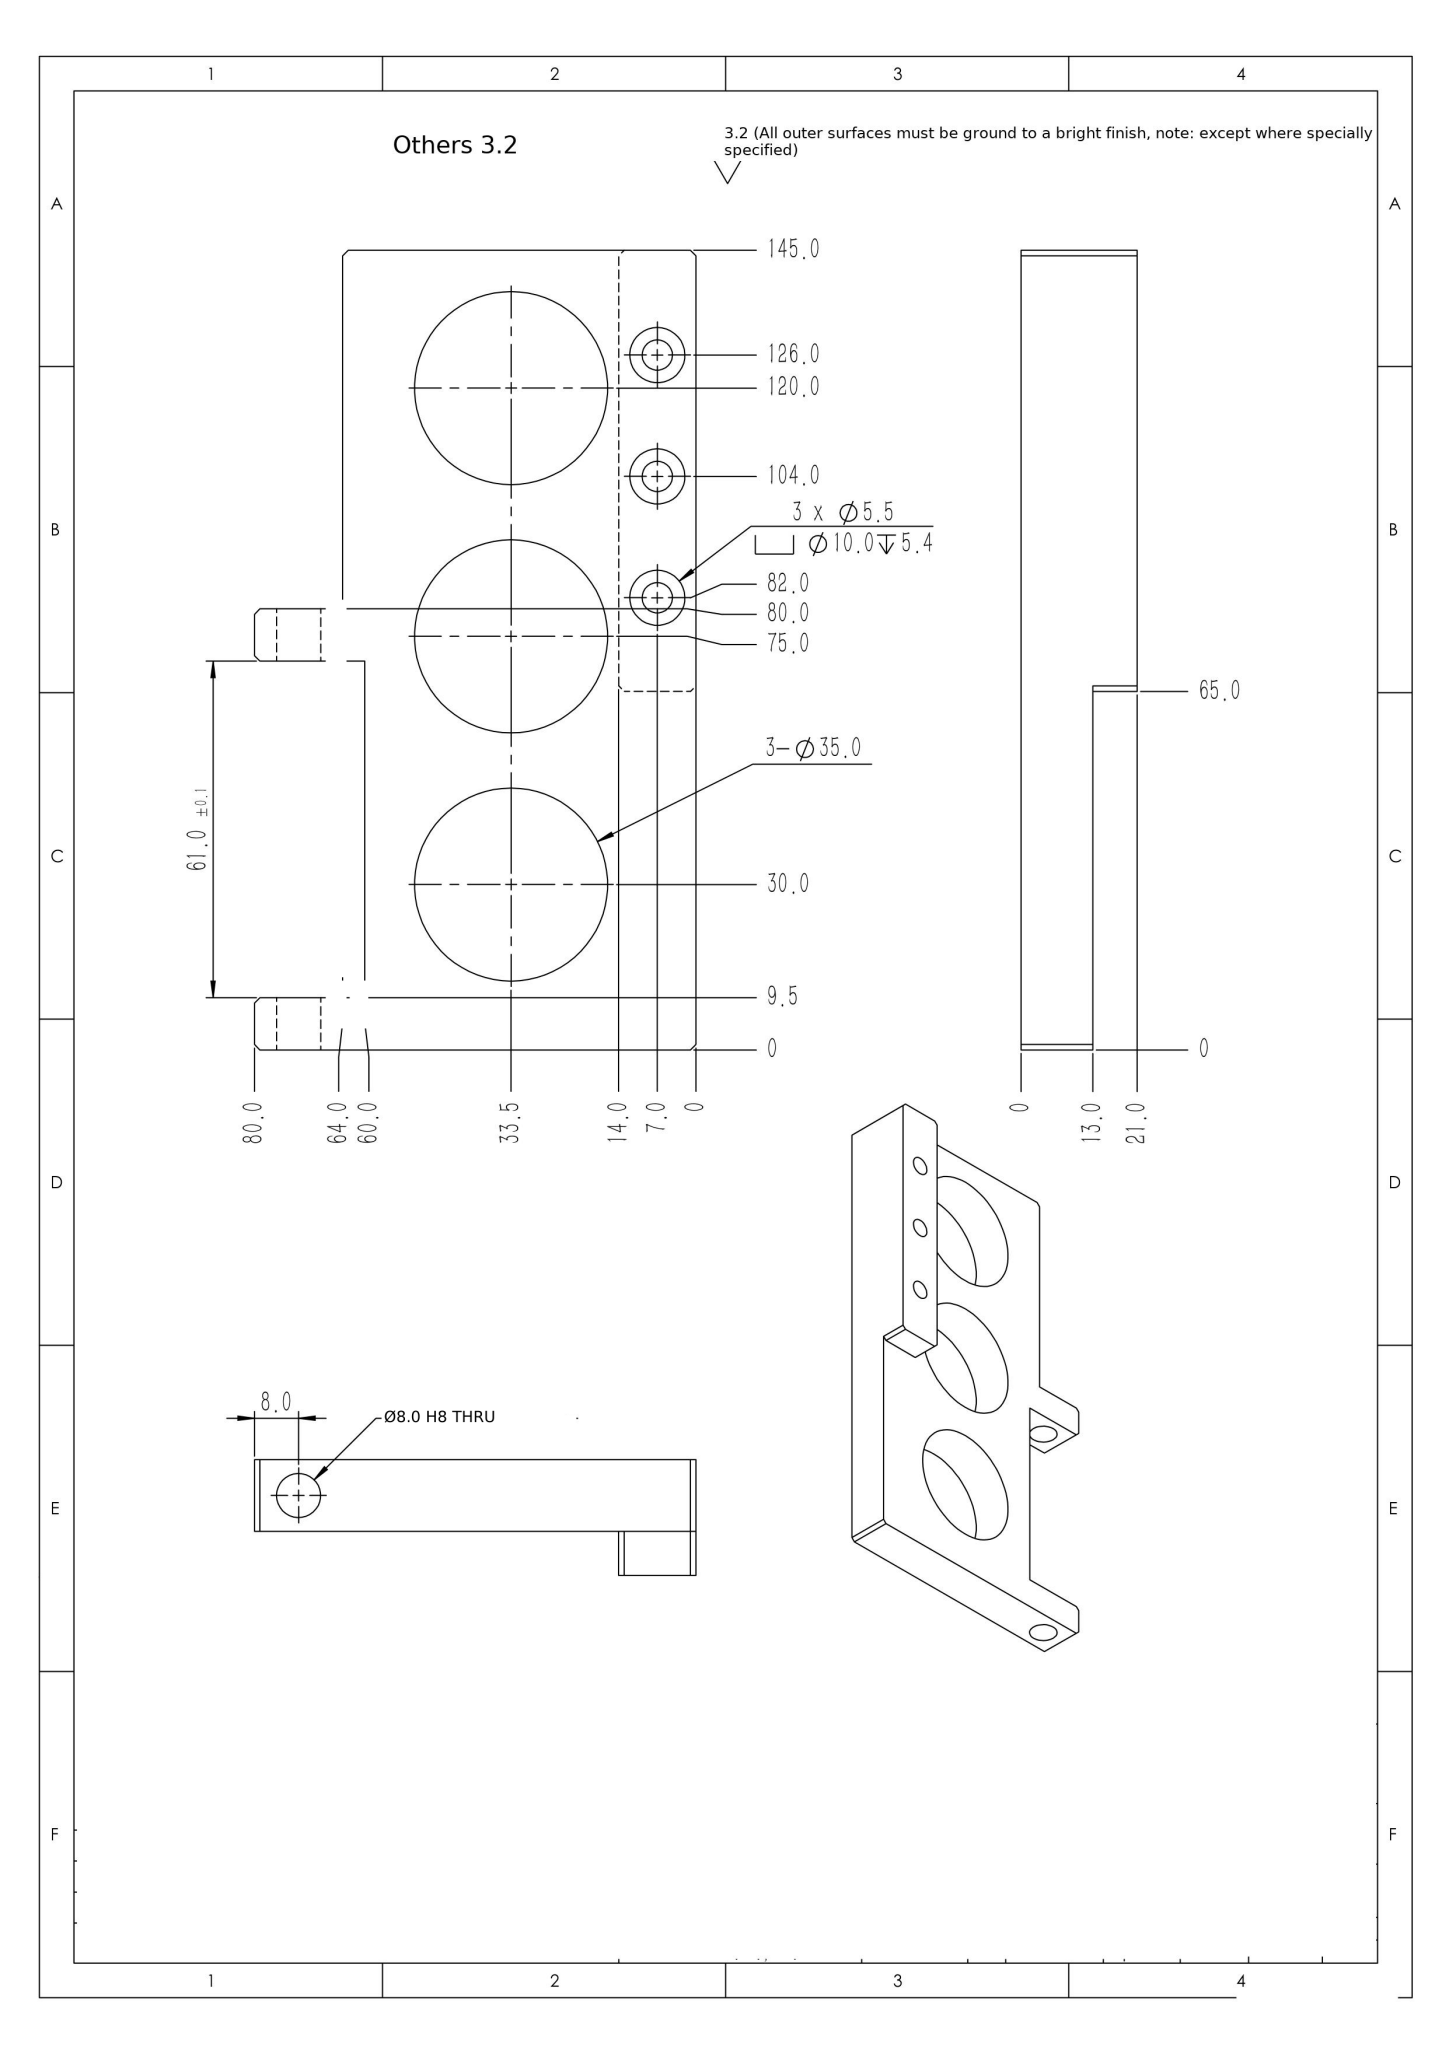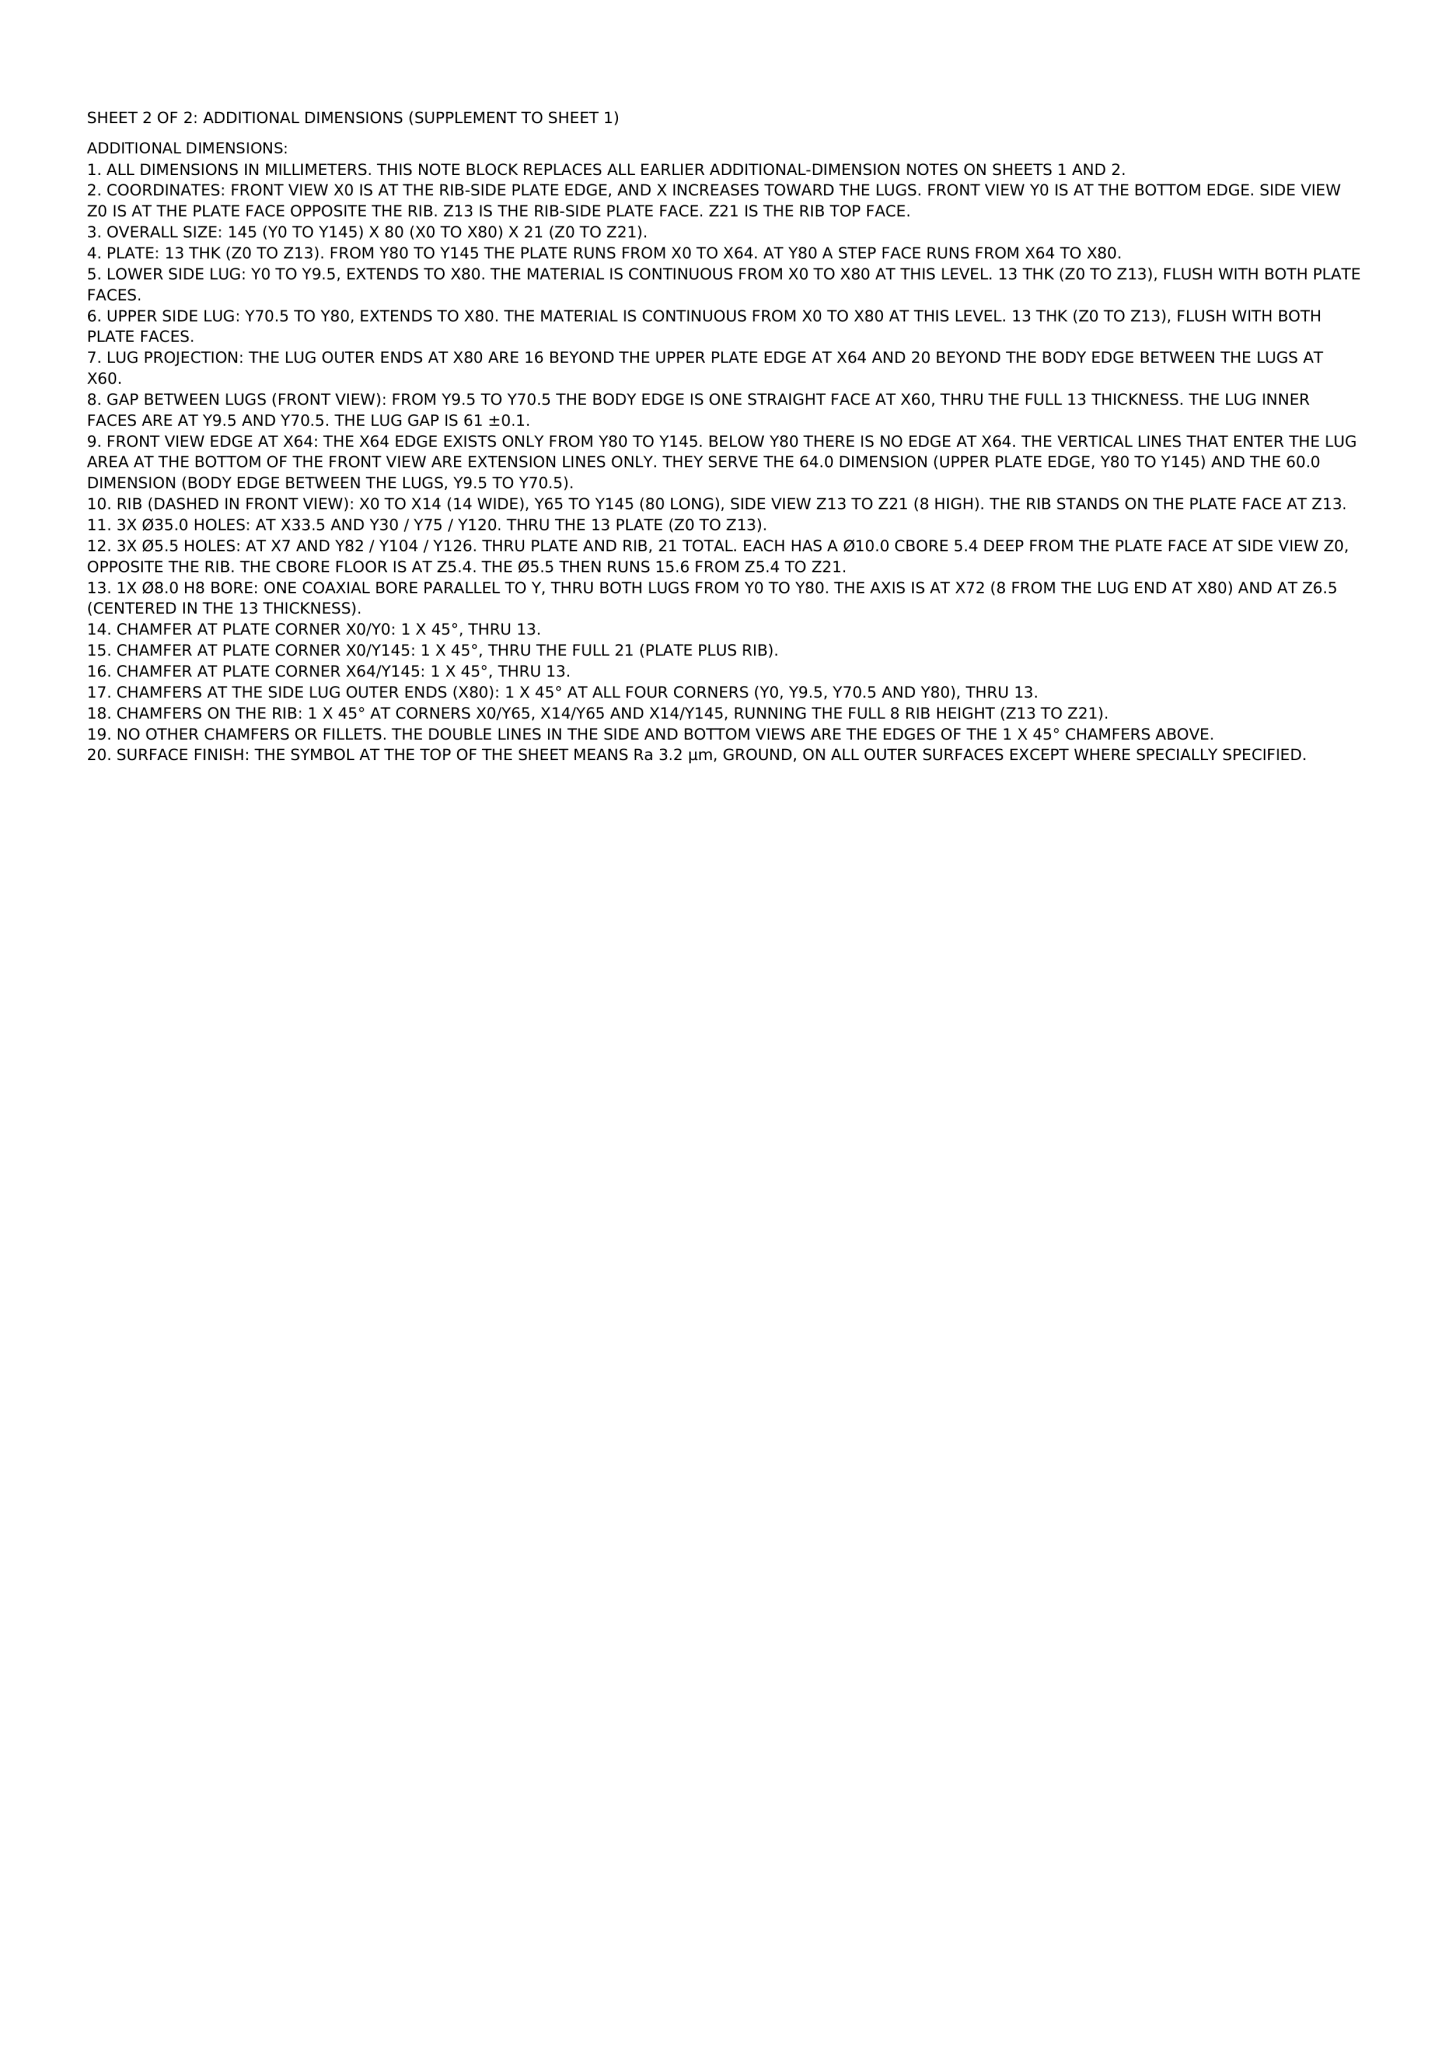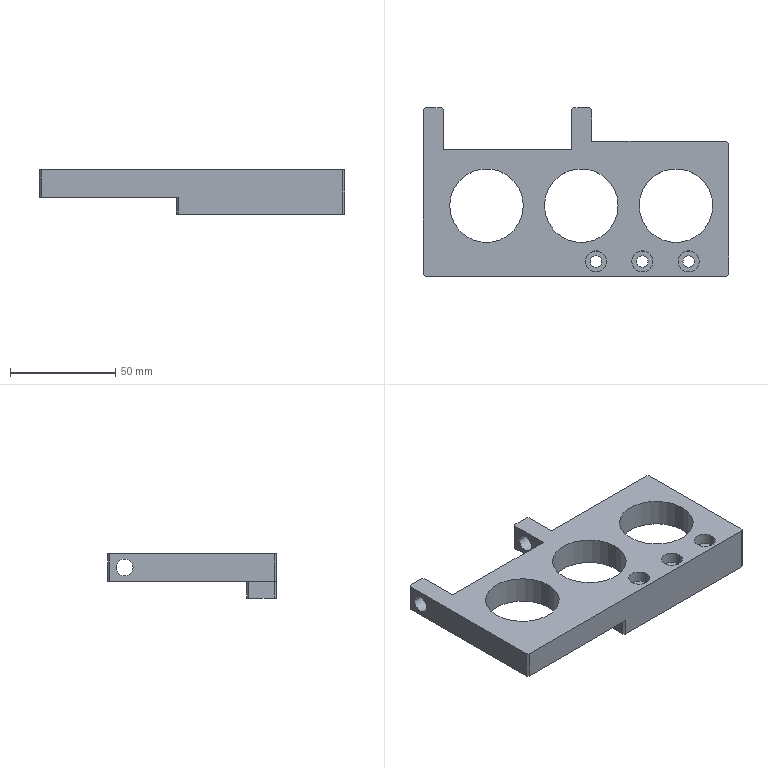Part | NX | mm | 1 solid | 50 faces | box 145 x 80 x 21 mm | volume 89457 mm3 | plane 28 | cylinder 22 | commonest cylinder face diameters 35 x6 10 x6 5.5 x6 8 x4